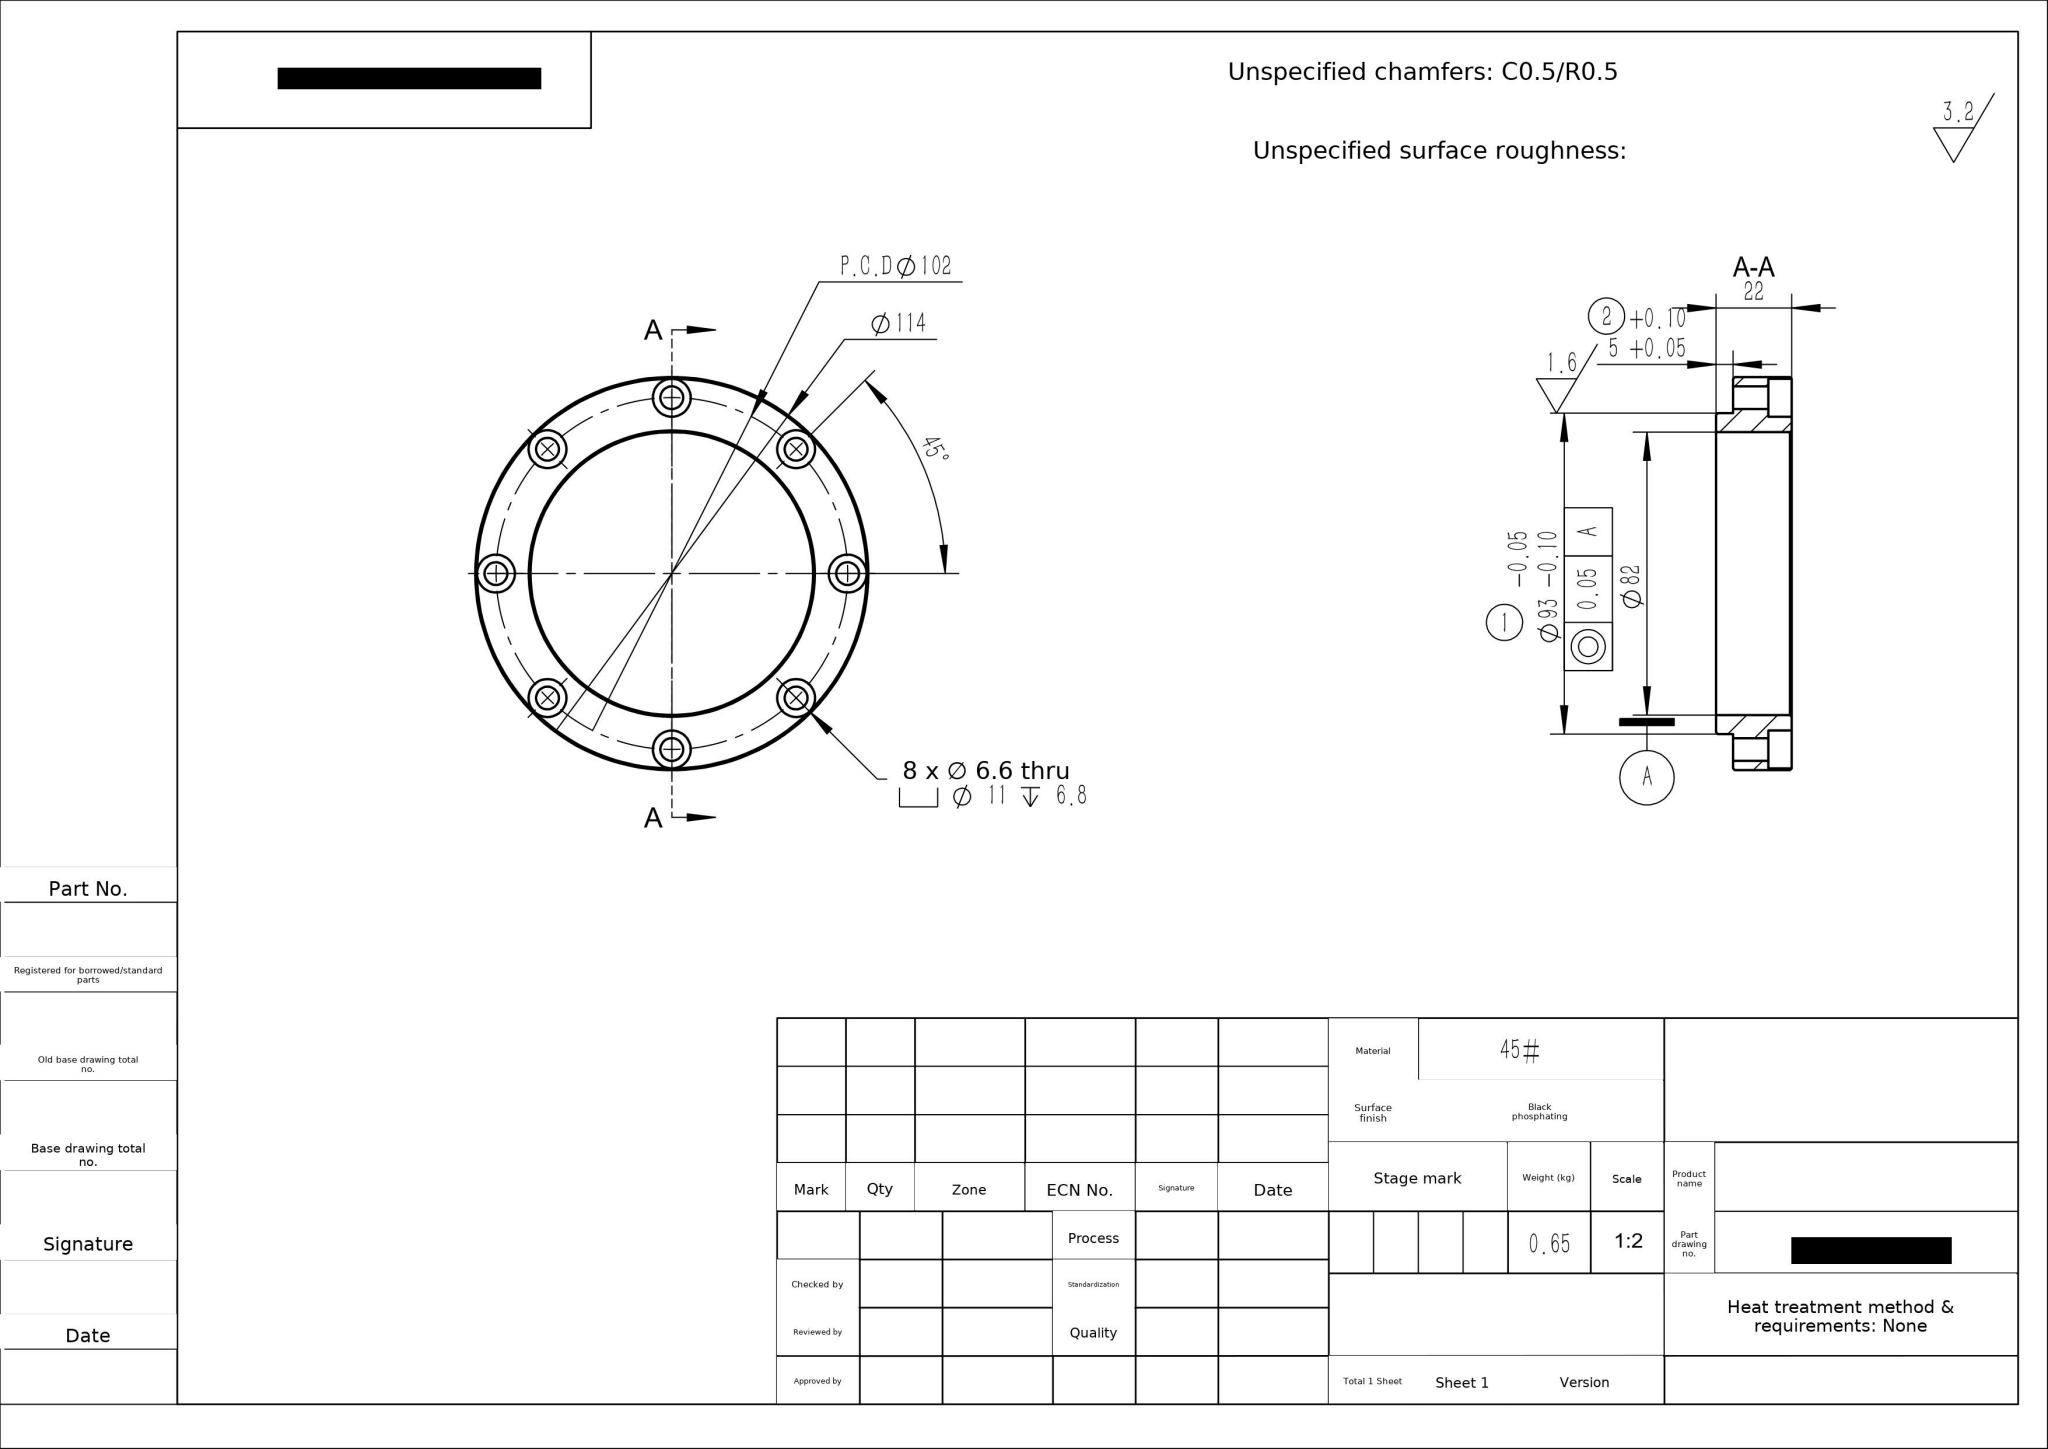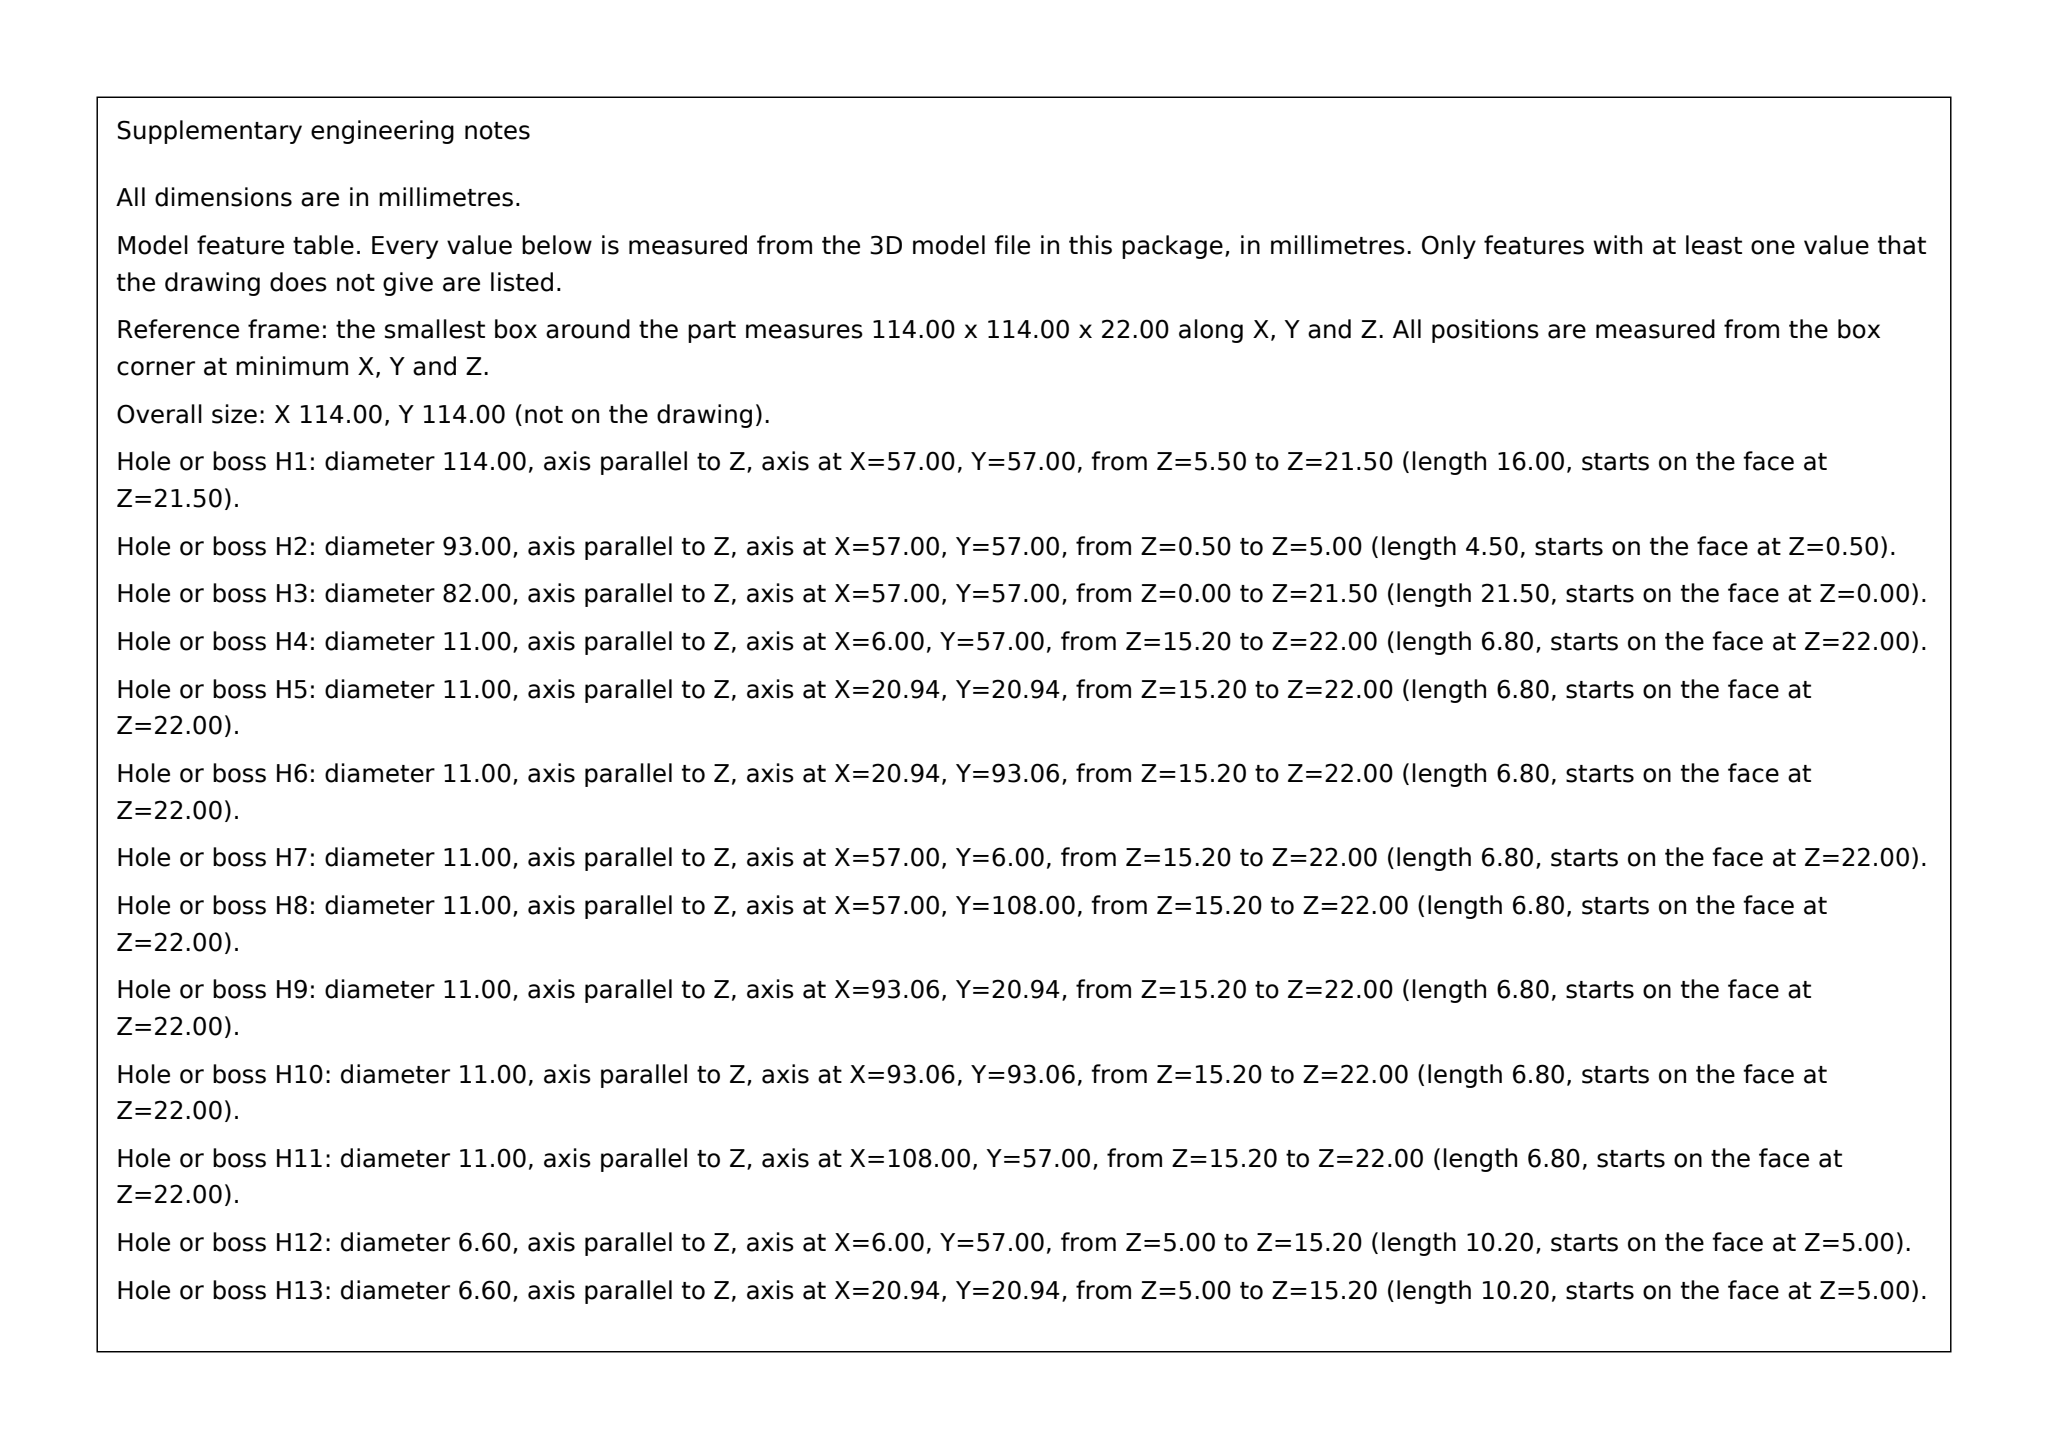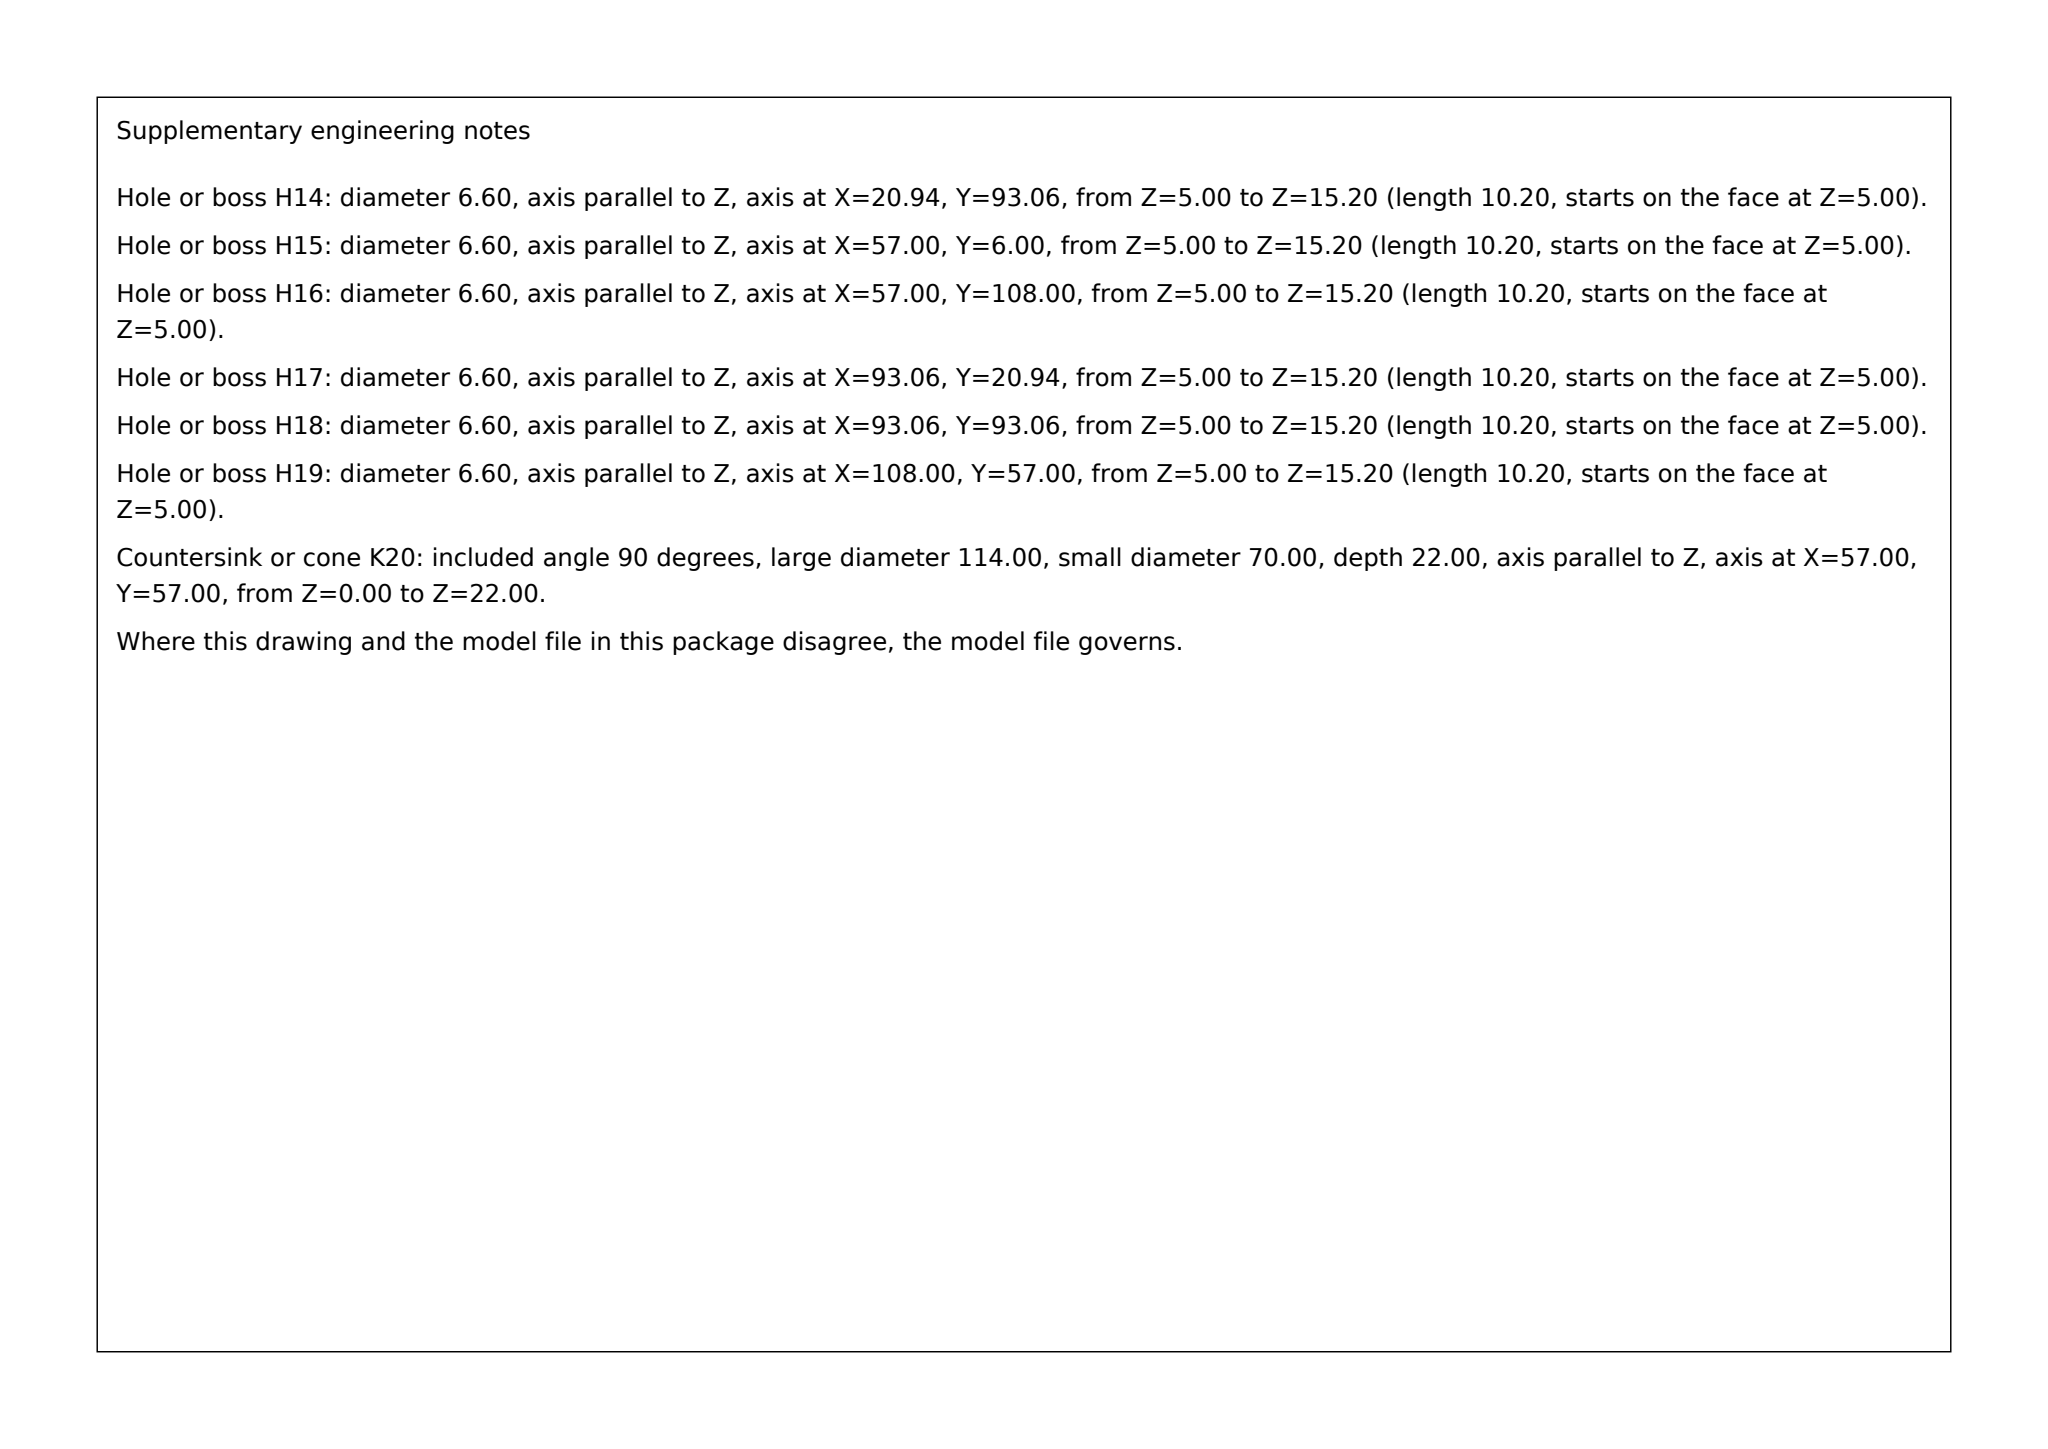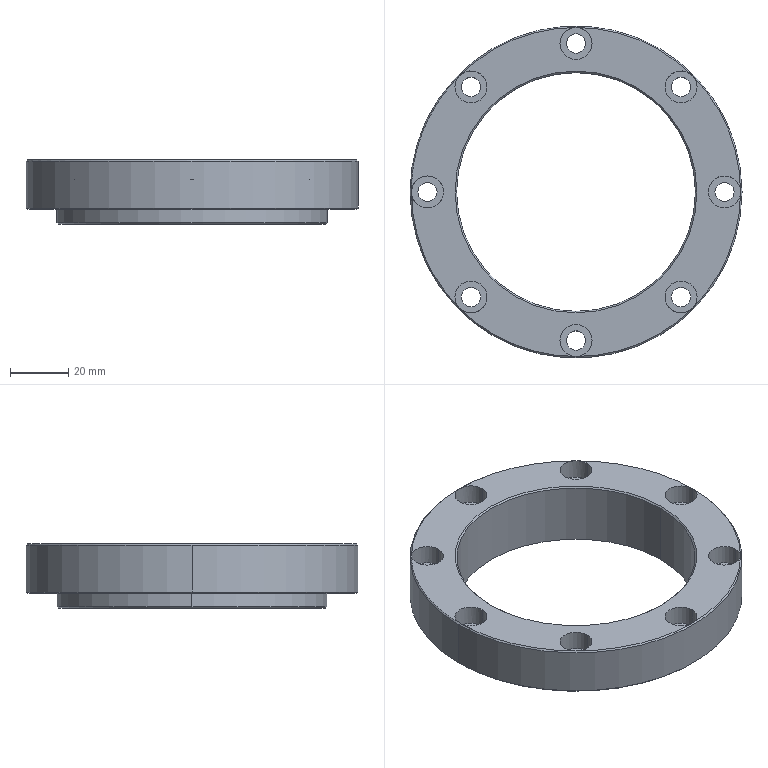Part | SolidWorks | mm | material 45# | 1 solid | 57 faces | box 114 x 114 x 22 mm | volume 83182 mm3 | cylinder 38 | plane 11 | cone 8 | commonest cylinder face diameters 11 x16 6.6 x16 82 x2 93 x2 114 x2
build123d program:
from build123d import *

# Parameters (mm, degrees)
SKETCH1_R                                            = 57
BOSS_EXTRUDE1_DEPTH                                  = 17
CHAMFER1_SIZE                                        = 0.5
SKETCH2_R                                            = 46.5
BOSS_EXTRUDE2_DEPTH                                  = 5
CHAMFER2_SIZE                                        = 0.5
SKETCH3_R                                            = 41
CUT_EXTRUDE1_DEPTH                                   = 84.558
HOLE_SIZE_ACCORDING_TO_TYPE_1_OF_HEXAGON_D           = 6.6
HOLE_SIZE_ACCORDING_TO_TYPE_1_OF_HEXAGON_CBORE_D     = 11
HOLE_SIZE_ACCORDING_TO_TYPE_1_OF_HEXAGON_CBORE_DEPTH = 6.8
CIRPATTERN1_COUNT                                    = 8
CHAMFER3_SIZE                                        = 0.5


with BuildPart() as part:
    # Sketch1 → Boss-Extrude1 (new body)
    with BuildSketch(Plane.XY):
        Circle(SKETCH1_R)
    extrude(amount=BOSS_EXTRUDE1_DEPTH)

    # Chamfer1
    chamfer1_edges = [part.edges().sort_by_distance(p)[0] for p in [
        (-57, 0, 0),
        (-57, 0, 17),
    ]]
    chamfer(chamfer1_edges, length=CHAMFER1_SIZE)

    # Sketch2 → Boss-Extrude2 (add)
    with BuildSketch(Plane(origin=(0, 0, 0), x_dir=(-1, 0, 0), z_dir=(0, 0, -1))):
        Circle(SKETCH2_R)
    extrude(amount=BOSS_EXTRUDE2_DEPTH)

    # Chamfer2
    chamfer2_edges = [part.edges().sort_by_distance(p)[0] for p in [
        (46.5, 0, -5),
    ]]
    chamfer(chamfer2_edges, length=CHAMFER2_SIZE)

    # Sketch3 → Cut-Extrude1 (cut, through all)
    with BuildSketch(Plane.XY.offset(17)):
        Circle(SKETCH3_R)
    extrude(amount=-CUT_EXTRUDE1_DEPTH, mode=Mode.SUBTRACT)

    # Hole Size_According to_Type 1 of Hexagon (through all)
    with Locations(Plane.XY.offset(17)):
        with Locations((0, 51)):
            hole_size_according_to_type_1_of_hexagon = CounterBoreHole(HOLE_SIZE_ACCORDING_TO_TYPE_1_OF_HEXAGON_D / 2, HOLE_SIZE_ACCORDING_TO_TYPE_1_OF_HEXAGON_CBORE_D / 2, HOLE_SIZE_ACCORDING_TO_TYPE_1_OF_HEXAGON_CBORE_DEPTH)

    # CirPattern1: Hole Size_According to_Type 1 of Hexagon ×8 about axis
    cirpattern1_axis = Axis((0, 0, 0), (0, 0, 1))
    for i in range(1, CIRPATTERN1_COUNT):
        add(hole_size_according_to_type_1_of_hexagon.rotate(cirpattern1_axis, i * 360 / CIRPATTERN1_COUNT), mode=Mode.SUBTRACT)

    # Chamfer3
    chamfer3_edges = [part.edges().sort_by_distance(p)[0] for p in [
        (-41, 0, 17),
    ]]
    chamfer(chamfer3_edges, length=CHAMFER3_SIZE)


solid = part.part